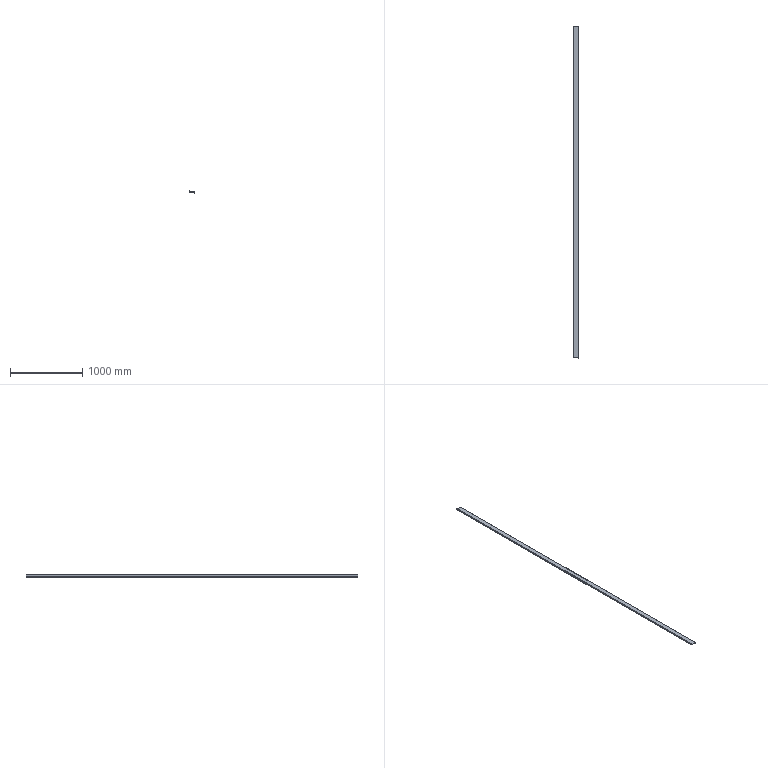Component | NX | 35_1 | 1 solid | 10 faces | volume 807300 mm3 | plane 10